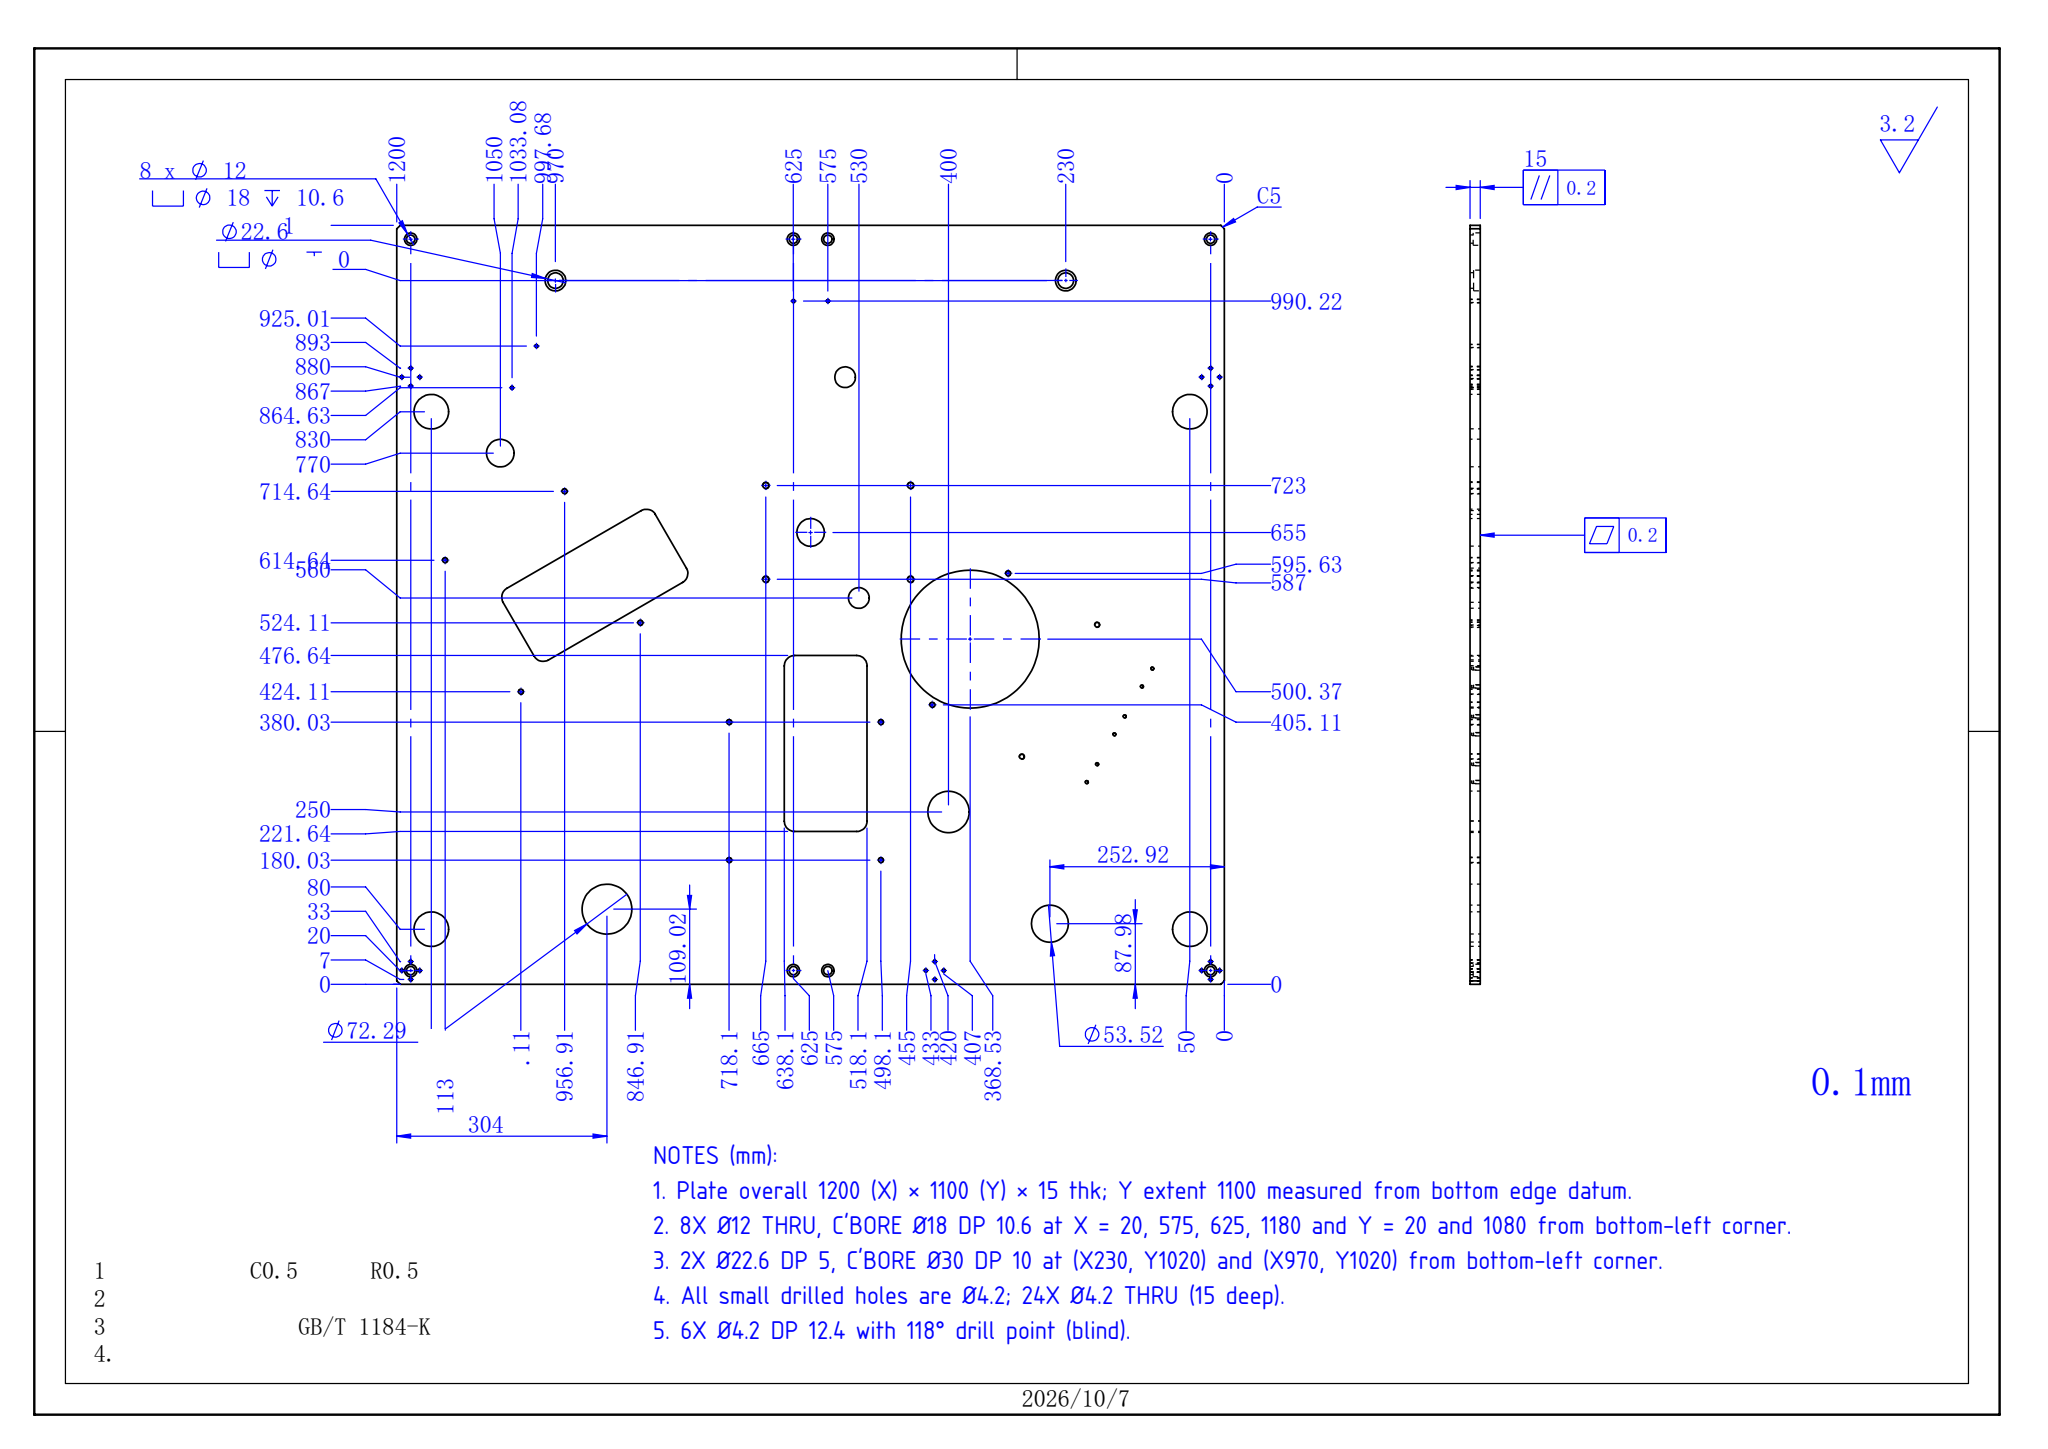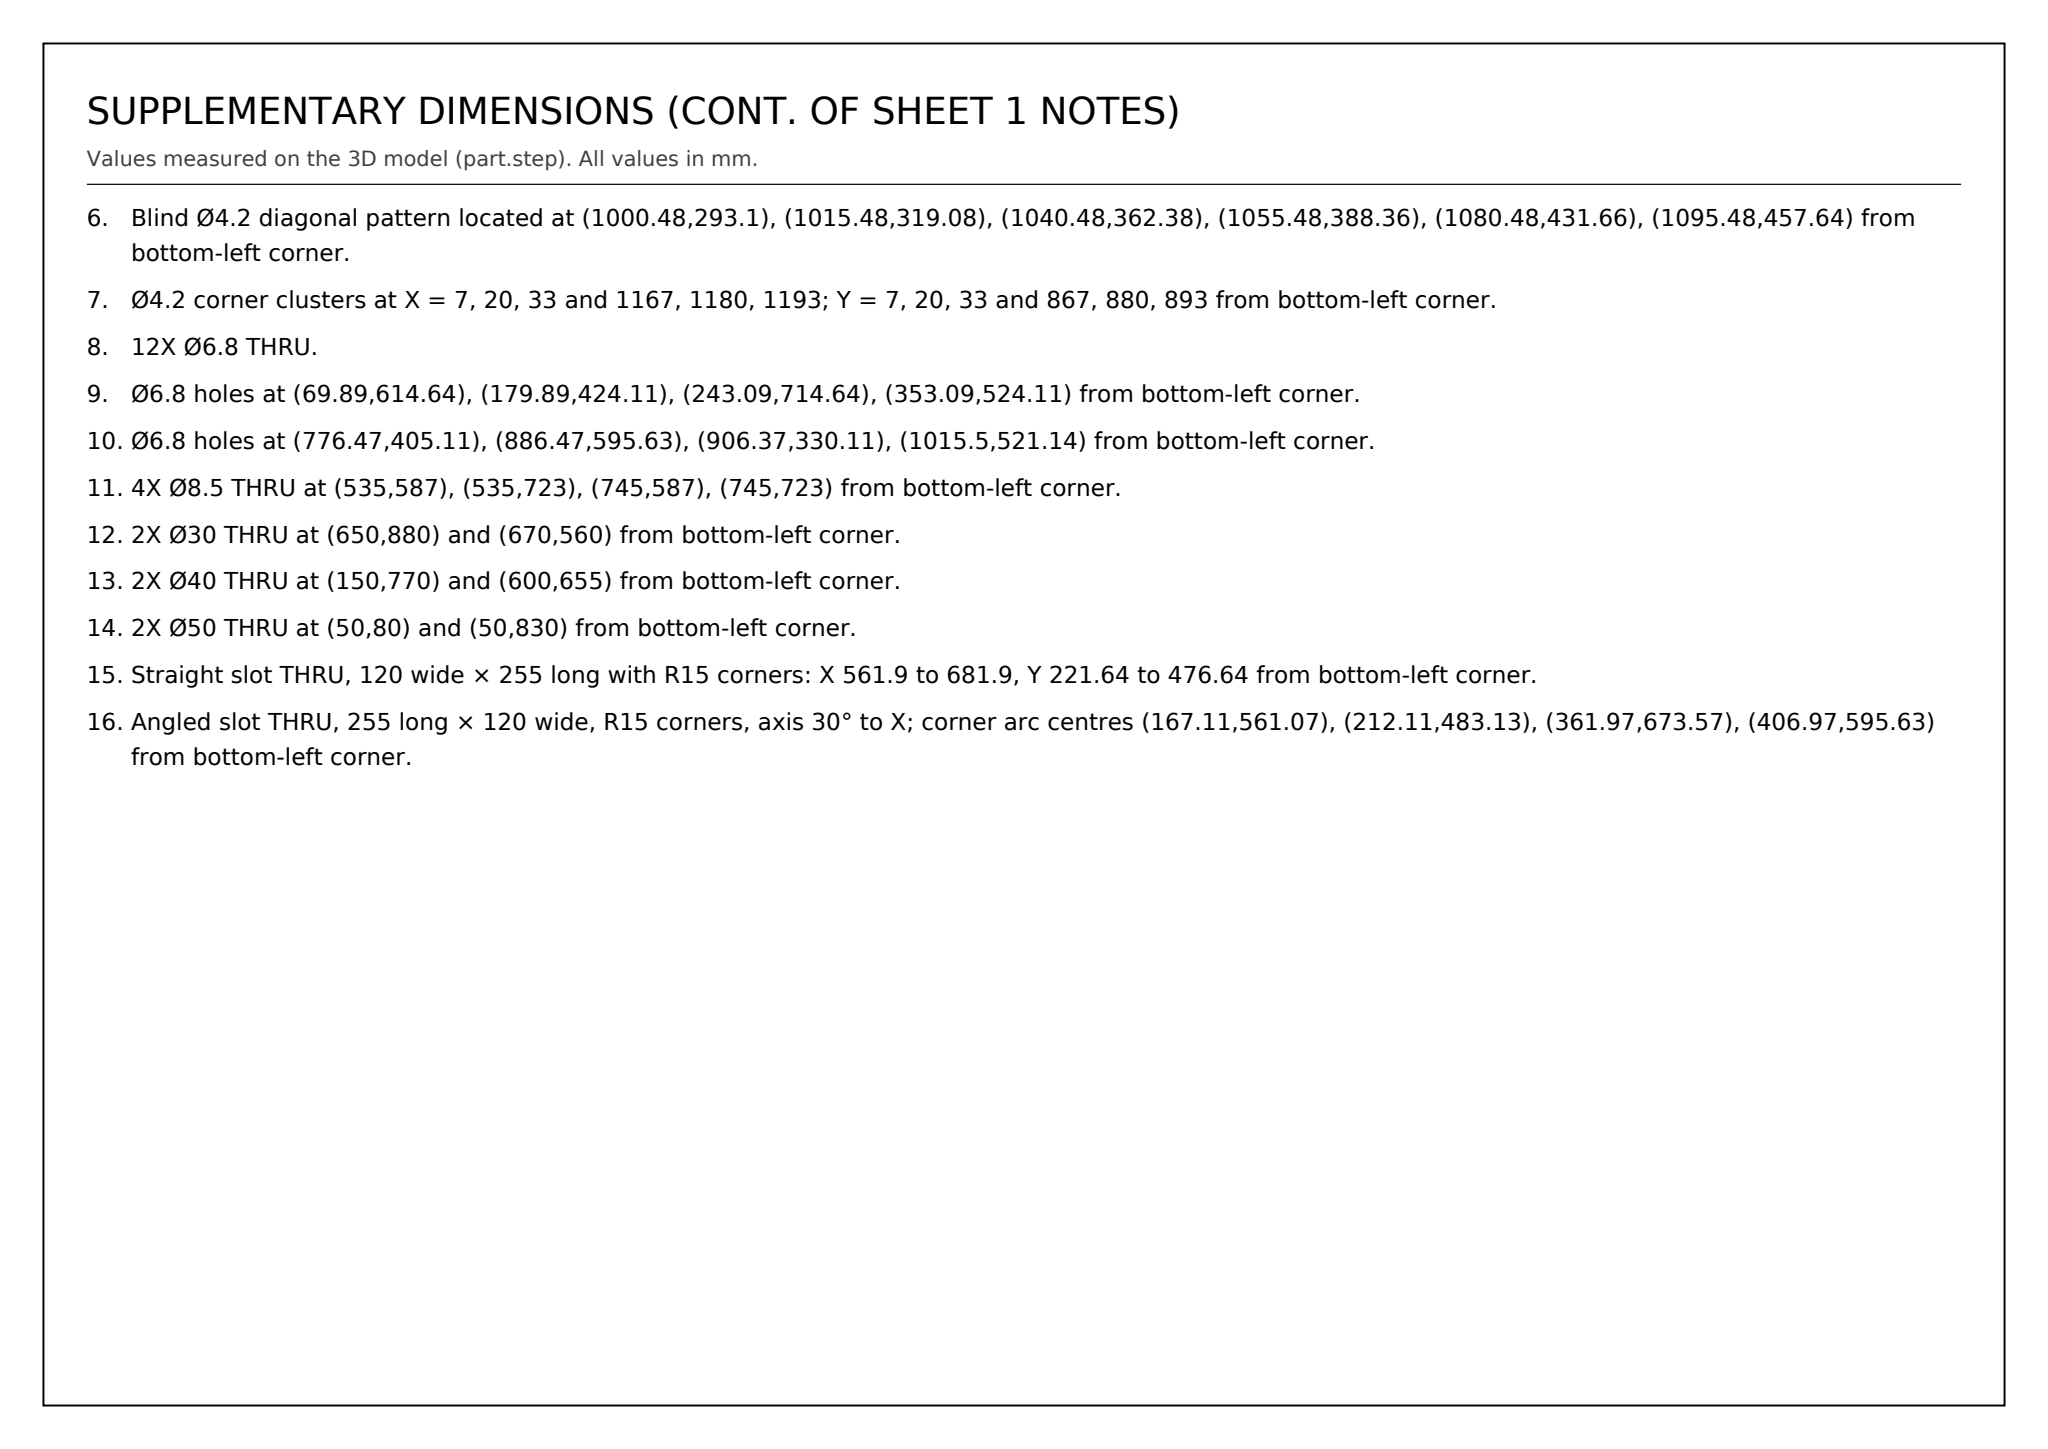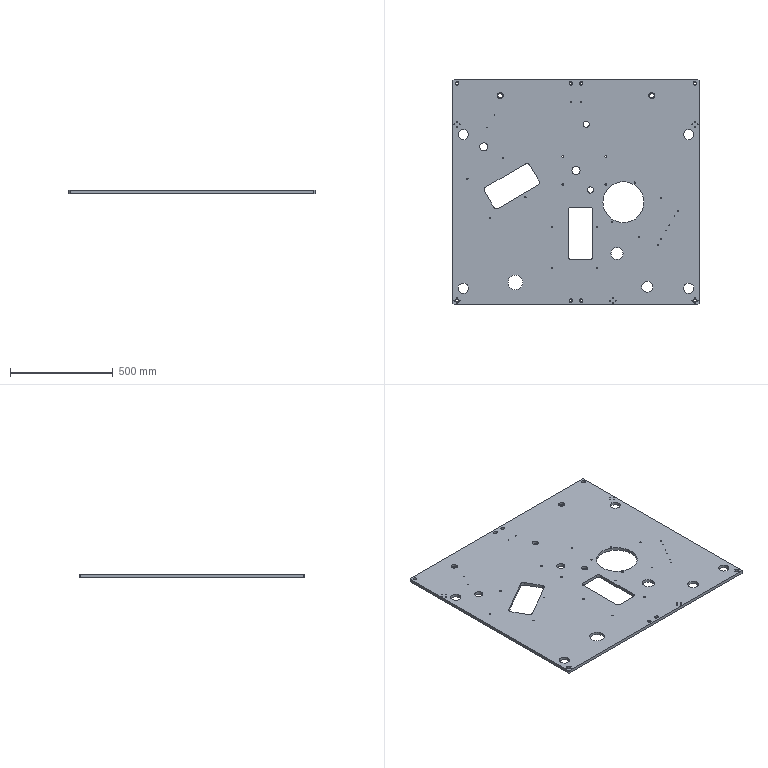Part | SolidWorks | mm | 1 solid | 204 faces | box 1200 x 1100 x 15 mm | volume 18041664 mm3 | cylinder 164 | plane 28 | cone 12 | commonest cylinder face diameters 4.2 x60 6.8 x24 30 x16 18 x16 12 x16 50 x8 8.5 x8 40 x4
Drawing notes:
Plate overall 1200 (X) × 1100 (Y) × 15 thk; Y extent 1100 measured from bottom edge datum. | from the solid: bbox_xyz [1200.0, 1100.0, 15.0]
8X Ø12 THRU, C'BORE Ø18 DP 10.6 at X = 20, 575, 625, 1180 and Y = 20 and 1080 from bottom-left corner. | from the solid: cylinders dia 12.0 len 4.4 and dia 18.0 len 10.6 at (20/575/625/1180, 20 and 1080)
2X Ø22.6 DP 5, C'BORE Ø30 DP 10 at (X230, Y1020) and (X970, Y1020) from bottom-left corner. | from the solid: cylinders dia 22.6 len 5.0 and dia 30.0 len 10.0 at [230,1020] and [970,1020]
All small drilled holes are Ø4.2; 24X Ø4.2 THRU (15 deep). | from the solid: cylinders dia 4.2 length 15.0 (24 positions)
6X Ø4.2 DP 12.4 with 118° drill point (blind). | from the solid: cylinders dia 4.2 length 12.4 (6 positions); cones [118.0, 4.2]
Blind Ø4.2 diagonal pattern located at (1000.48,293.1), (1015.48,319.08), (1040.48,362.38), (1055.48,388.36), (1080.48,431.66), (1095.48,457.64) from bottom-left corner. | from the solid: cylinders dia 4.2 len 12.4 positions
Ø4.2 corner clusters at X = 7, 20, 33 and 1167, 1180, 1193; Y = 7, 20, 33 and 867, 880, 893 from bottom-left corner. | from the solid: cylinders dia 4.2 len 15 at [7,20],[20,7],[20,33],[33,20],[1167,20],[1180,7],[1180,33],[1193,20],[7,880],[20,867],[20,893],[33,880],[1167,880],[1180,867],[1180,893],[1193,880]
12X Ø6.8 THRU. | from the solid: cylinders dia 6.8 length 15.0 (12 positions)
Ø6.8 holes at (69.89,614.64), (179.89,424.11), (243.09,714.64), (353.09,524.11) from bottom-left corner. | from the solid: cylinders dia 6.8 at [69.89,614.64],[179.89,424.11],[243.09,714.64],[353.09,524.11]
Ø6.8 holes at (776.47,405.11), (886.47,595.63), (906.37,330.11), (1015.5,521.14) from bottom-left corner. | from the solid: cylinders dia 6.8 at [776.47,405.11],[886.47,595.63],[906.37,330.11],[1015.5,521.14]
4X Ø8.5 THRU at (535,587), (535,723), (745,587), (745,723) from bottom-left corner. | from the solid: cylinders dia 8.5 length 15.0
2X Ø30 THRU at (650,880) and (670,560) from bottom-left corner. | from the solid: cylinders dia 30.0 length 15.0 at [650,880] and [670,560]
2X Ø40 THRU at (150,770) and (600,655) from bottom-left corner. | from the solid: cylinders dia 40.0 length 15.0
2X Ø50 THRU at (50,80) and (50,830) from bottom-left corner. | from the solid: cylinders dia 50.0 length 15.0
Straight slot THRU, 120 wide × 255 long with R15 corners: X 561.9 to 681.9, Y 221.64 to 476.64 from bottom-left corner. | from the solid: axis_planes x 561.9/681.9, y 221.64/476.64; dia 30 corner cylinders at [576.9,236.64],[576.9,461.64],[666.9,236.64],[666.9,461.64]
Angled slot THRU, 255 long × 120 wide, R15 corners, axis 30° to X; corner arc centres (167.11,561.07), (212.11,483.13), (361.97,673.57), (406.97,595.63) from bottom-left corner. | from the solid: dia 30.0 len 15.0 count 1 cylinders at [167.11,561.07],[212.11,483.13],[361.97,673.57],[406.97,595.63]
build123d program:
from build123d import *

# Parameters (mm, degrees)
SKETCH1_W                                        = 1200
SKETCH1_H                                        = 1100
BOSS_EXTRUDE1_DEPTH                              = 15
M10_HEX_SOCKET_HEAD_CAP_SCREW_CBORE1_D           = 12
M10_HEX_SOCKET_HEAD_CAP_SCREW_CBORE1_CBORE_D     = 18
M10_HEX_SOCKET_HEAD_CAP_SCREW_CBORE1_CBORE_DEPTH = 10.6
LPATTERN1_COUNT                                  = 2
LPATTERN1_PITCH                                  = 1060
CHAMFER1_SIZE                                    = 5
M5_TAPPED_HOLE1_D                                = 4.2
SKETCH7_R                                        = 11.3
CUT_EXTRUDE1_DEPTH                               = 15
SKETCH8_R                                        = 15
CUT_EXTRUDE2_DEPTH                               = 10
LPATTERN2_COUNT                                  = 2
LPATTERN2_PITCH                                  = 740
SKETCH9_R                                        = 20
CUT_EXTRUDE3_DEPTH                               = 1628.951
M5_TAPPED_HOLE2_D                                = 4.2
CUT_EXTRUDE4_DEPTH                               = 1628.951
SKETCH14_R                                       = 100
CUT_EXTRUDE5_DEPTH                               = 1628.951
M10_TAPPED_HOLE1_D                               = 8.5
FILLET1_R                                        = 15
M8_TAPPED_HOLE2_D                                = 6.8
M8_TAPPED_HOLE3_D                                = 6.8
SKETCH23_R                                       = 20
SKETCH23_R_2                                     = 15
SKETCH23_R_3                                     = 30
CUT_EXTRUDE6_DEPTH                               = 1628.951
SKETCH24_R                                       = 25
CUT_EXTRUDE7_DEPTH                               = 1628.951
SKETCH25_R                                       = 15
CUT_EXTRUDE8_DEPTH                               = 1628.951
M5_TAPPED_HOLE3_D                                = 4.2
M5_TAPPED_HOLE3_DEPTH                            = 12.4
M5_TAPPED_HOLE3_TIP                              = 1.262
M8_TAPPED_HOLE4_D                                = 6.8
SKETCH30_R                                       = 36.147
SKETCH30_R_2                                     = 26.758
CUT_EXTRUDE9_DEPTH                               = 50


with BuildPart() as part:
    # Sketch1 → Boss-Extrude1 (new body)
    with BuildSketch(Plane.XY):
        with Locations((600, 550)):
            Rectangle(SKETCH1_W, SKETCH1_H)
    extrude(amount=BOSS_EXTRUDE1_DEPTH)

    # M10 Hex Socket Head Cap Screw CBORE1 (through all)
    with Locations(Plane.XY.offset(15)):
        with Locations((1180, 20), (20, 20), (575, 20), (625, 20)):
            m10_hex_socket_head_cap_screw_cbore1 = CounterBoreHole(M10_HEX_SOCKET_HEAD_CAP_SCREW_CBORE1_D / 2, M10_HEX_SOCKET_HEAD_CAP_SCREW_CBORE1_CBORE_D / 2, M10_HEX_SOCKET_HEAD_CAP_SCREW_CBORE1_CBORE_DEPTH)

    # LPattern1: M10 Hex Socket Head Cap Screw CBORE1 ×2
    with Locations(*[(0, i * LPATTERN1_PITCH, 0) for i in range(1, LPATTERN1_COUNT)]):
        add(m10_hex_socket_head_cap_screw_cbore1, mode=Mode.SUBTRACT)

    # Chamfer1
    chamfer1_edges = [part.edges().sort_by_distance(p)[0] for p in [
        (0, 1100, 7.5),
        (1200, 1100, 7.5),
        (1200, 0, 7.5),
        (0, 0, 7.5),
    ]]
    chamfer(chamfer1_edges, length=CHAMFER1_SIZE)

    # M5 Tapped Hole1 (through all)
    with Locations(Plane.XY.offset(15)):
        with Locations((1167, 20), (1180, 7), (1193, 20), (1180, 33), (1167, 880), (1180, 893), (1180, 867), (1193, 880), (767, 20), (780, 33), (780, 7), (793, 20), (7, 20), (20, 33), (20, 7), (33, 20), (7, 880), (20, 893), (20, 867), (33, 880)):
            Hole(M5_TAPPED_HOLE1_D / 2)

    # Sketch7 → Cut-Extrude1 (cut)
    with BuildSketch(Plane.XY.offset(15)):
        with Locations((970, 1020)):
            Circle(SKETCH7_R)
    cut_extrude1 = extrude(amount=-CUT_EXTRUDE1_DEPTH, mode=Mode.SUBTRACT)

    # Sketch8 → Cut-Extrude2 (cut)
    with BuildSketch(Plane.XY.offset(15)):
        with Locations((970, 1020)):
            Circle(SKETCH8_R)
    cut_extrude2 = extrude(amount=-CUT_EXTRUDE2_DEPTH, mode=Mode.SUBTRACT)

    # LPattern2: Cut-Extrude1, Cut-Extrude2 ×2
    with Locations(*[(-i * LPATTERN2_PITCH, 0, 0) for i in range(1, LPATTERN2_COUNT)]):
        add(cut_extrude1, mode=Mode.SUBTRACT)
        add(cut_extrude2, mode=Mode.SUBTRACT)

    # Sketch9 → Cut-Extrude3 (cut, through all)
    with BuildSketch(Plane.XY.offset(15)):
        with Locations((600, 655)):
            Circle(SKETCH9_R)
    extrude(amount=-CUT_EXTRUDE3_DEPTH, mode=Mode.SUBTRACT)

    # M5 Tapped Hole2 (through all)
    with Locations(Plane.XY.offset(15)):
        with Locations((625, 990.224), (575, 990.224), (166.917, 864.626), (202.325, 925.013)):
            Hole(M5_TAPPED_HOLE2_D / 2)

    # Sketch13 → Cut-Extrude4 (cut, through all)
    with BuildSketch(Plane.XY.offset(15)):
        with BuildLine():
            Line((561.9, 236.642), (561.9, 476.642))
            Line((561.9, 476.642), (681.9, 476.642))
            Line((681.9, 476.642), (681.9, 236.642))
            ThreePointArc((681.9, 236.642), (677.507, 226.035), (666.9, 221.642))
            Line((666.9, 221.642), (576.9, 221.642))
            ThreePointArc((576.9, 221.642), (566.293, 226.035), (561.9, 236.642))
        make_face()
        with BuildLine():
            Line((159.61, 574.061), (367.456, 694.061))
            Line((367.456, 694.061), (427.456, 590.138))
            Line((427.456, 590.138), (219.61, 470.138))
            ThreePointArc((219.61, 470.138), (208.228, 468.64), (199.12, 475.629))
            Line((199.12, 475.629), (154.12, 553.571))
            ThreePointArc((154.12, 553.571), (152.621, 564.953), (159.61, 574.061))
        make_face()
    extrude(amount=-CUT_EXTRUDE4_DEPTH, mode=Mode.SUBTRACT)

    # Sketch14 → Cut-Extrude5 (cut, through all)
    with BuildSketch(Plane.XY.offset(15)):
        with Locations((831.471, 500.372)):
            Circle(SKETCH14_R)
    extrude(amount=-CUT_EXTRUDE5_DEPTH, mode=Mode.SUBTRACT)

    # M10 Tapped Hole1 (through all)
    with Locations(Plane.XY.offset(15)):
        with Locations((745, 723), (745, 587), (535, 723), (535, 587)):
            Hole(M10_TAPPED_HOLE1_D / 2)

    # Fillet1
    fillet1_edges = [part.edges().sort_by_distance(p)[0] for p in [
        (561.9, 476.642, 7.5),
        (681.9, 476.642, 7.5),
        (367.456, 694.061, 7.5),
        (427.456, 590.138, 7.5),
    ]]
    fillet(fillet1_edges, radius=FILLET1_R)

    # M8 Tapped Hole2 (through all)
    with Locations(Plane.XY.offset(15)):
        with Locations((701.9, 380.026), (701.9, 180.026), (481.9, 180.026), (481.9, 380.026), (353.092, 524.11), (179.887, 424.11), (69.887, 614.636), (243.092, 714.636)):
            Hole(M8_TAPPED_HOLE2_D / 2)

    # M8 Tapped Hole3 (through all)
    with Locations(Plane.XY.offset(15)):
        with Locations((886.471, 595.635), (776.471, 405.109)):
            Hole(M8_TAPPED_HOLE3_D / 2)

    # Sketch23 → Cut-Extrude6 (cut, through all)
    with BuildSketch(Plane.XY.offset(15)):
        with Locations((150, 770)):
            Circle(SKETCH23_R)
        with Locations((670, 560)):
            Circle(SKETCH23_R_2)
        with Locations((800, 250)):
            Circle(SKETCH23_R_3)
    extrude(amount=-CUT_EXTRUDE6_DEPTH, mode=Mode.SUBTRACT)

    # Sketch24 → Cut-Extrude7 (cut, through all)
    with BuildSketch(Plane.XY.offset(15)):
        with Locations((50, 830)):
            Circle(SKETCH24_R)
        with Locations((50, 80)):
            Circle(SKETCH24_R)
    cut_extrude7 = extrude(amount=-CUT_EXTRUDE7_DEPTH, mode=Mode.SUBTRACT)

    # Mirror1: Cut-Extrude7 across plane
    add(cut_extrude7.mirror(Plane(origin=(600, 0, 0), x_dir=(0, 0, 1), z_dir=(1, 0, 0))), mode=Mode.SUBTRACT)

    # Sketch25 → Cut-Extrude8 (cut, through all)
    with BuildSketch(Plane.XY.offset(15)):
        with Locations((650, 880)):
            Circle(SKETCH25_R)
    extrude(amount=-CUT_EXTRUDE8_DEPTH, mode=Mode.SUBTRACT)

    # M5 Tapped Hole3
    with Locations(Plane.XY.offset(15)):
        with Locations((1095.477, 457.644), (1080.477, 431.663), (1055.477, 388.362), (1040.477, 362.381), (1015.477, 319.08), (1000.477, 293.099)):
            Hole(M5_TAPPED_HOLE3_D / 2, depth=M5_TAPPED_HOLE3_DEPTH)
            with Locations((0, 0, -(M5_TAPPED_HOLE3_DEPTH + M5_TAPPED_HOLE3_TIP / 2))):  # 118° drill point
                Cone(0, M5_TAPPED_HOLE3_D / 2, M5_TAPPED_HOLE3_TIP, mode=Mode.SUBTRACT)

    # M8 Tapped Hole4 (through all)
    with Locations(Plane.XY.offset(15)):
        with Locations((906.375, 330.109), (1015.498, 521.141)):
            Hole(M8_TAPPED_HOLE4_D / 2)

    # Sketch30 → Cut-Extrude9 (cut)
    with BuildSketch(Plane.XY.offset(15)):
        with Locations((304.608, 109.022)):
            Circle(SKETCH30_R)
        with Locations((947.082, 87.982)):
            Circle(SKETCH30_R_2)
    extrude(amount=-CUT_EXTRUDE9_DEPTH, mode=Mode.SUBTRACT)


solid = part.part